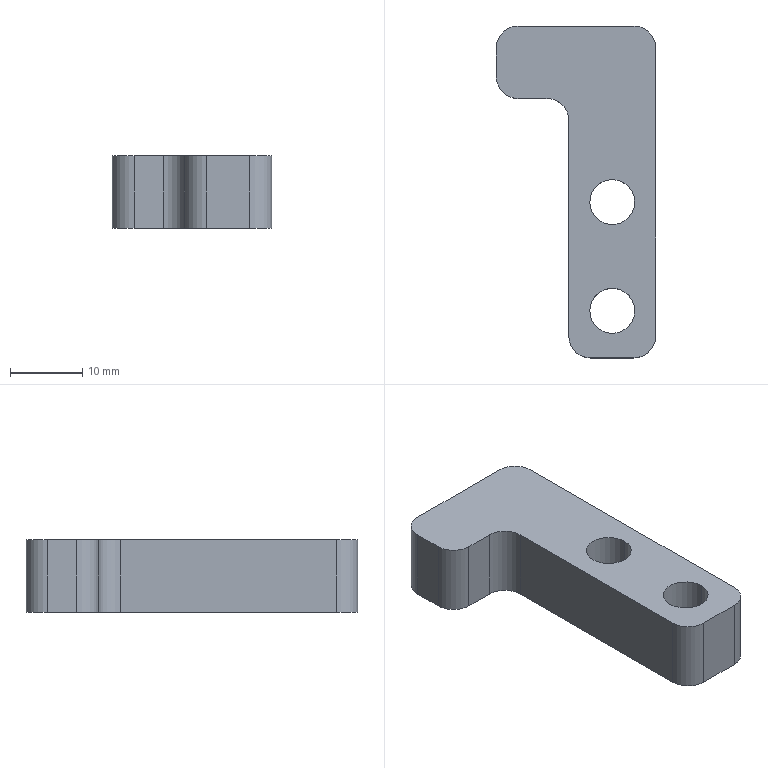CAM job | Mastercam | mm | 8 operations | part box 22 x 45.8 x 10
1. Facing | 23 - 63 平铣刀
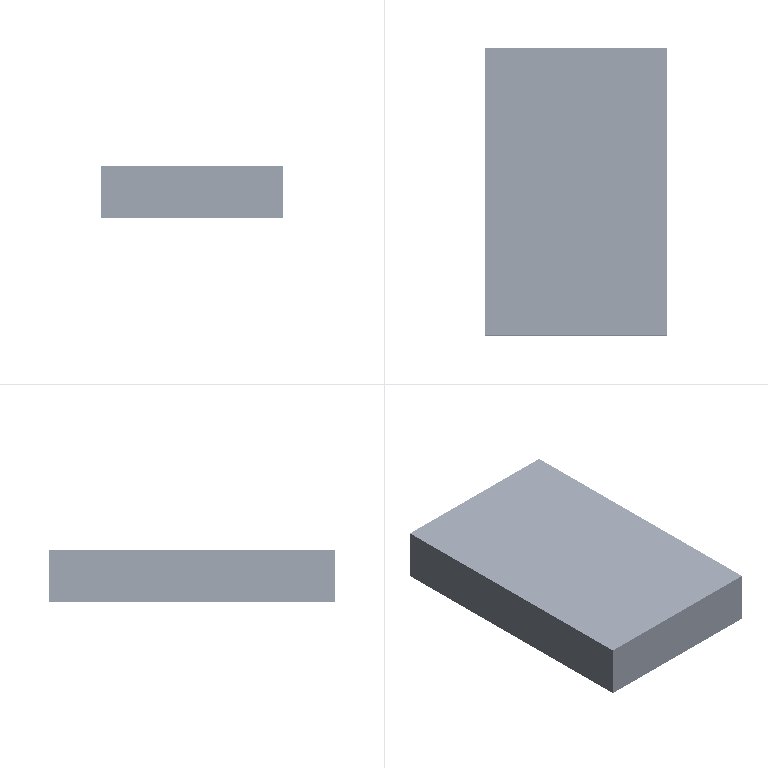2. 2D High Speed (2D Dynamic Mill) | 9 - 10 平铣刀
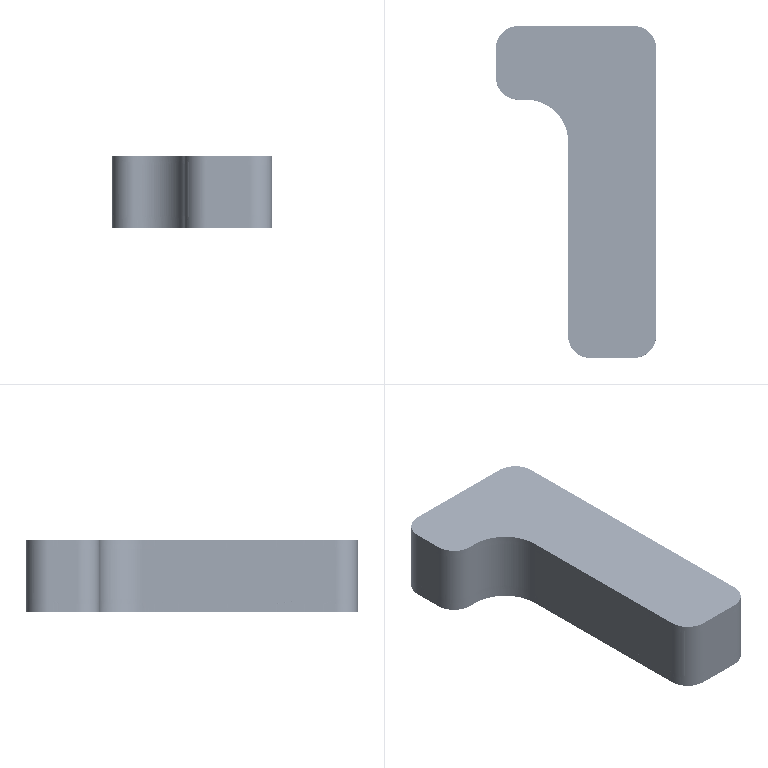3. Contour (Remachining) | 4 - 4 平铣刀
4. Contour (2D) | 4 - 4 平铣刀
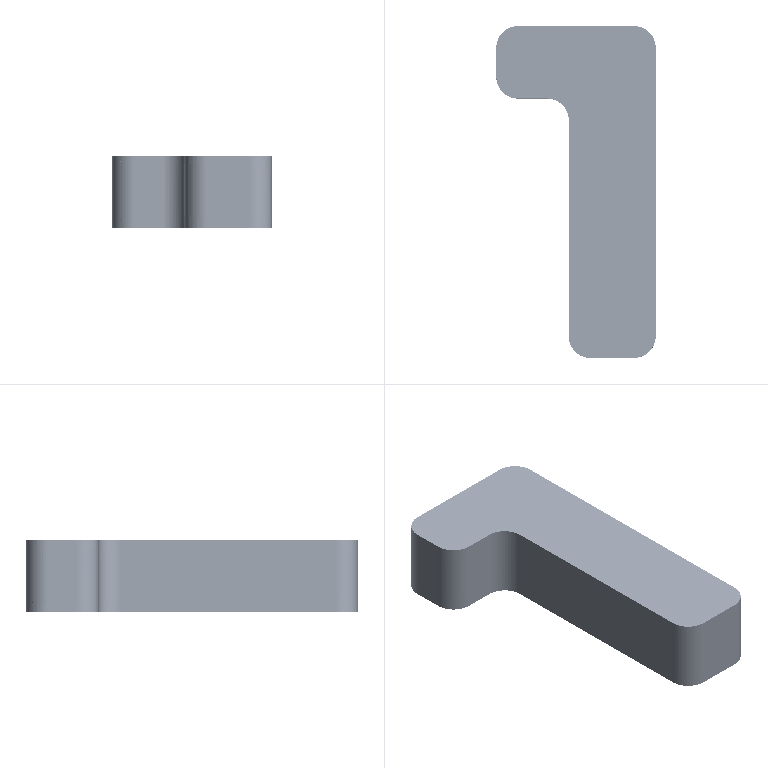5. Drill/Counterbore | 5 - 4 倒角刀
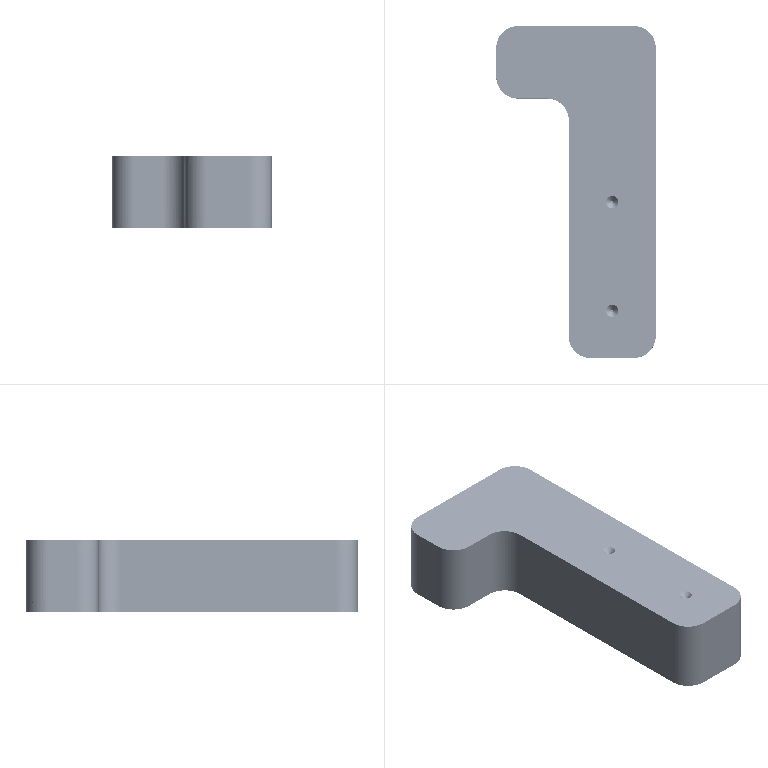6. Contour (2D chamfer) | 5 - 4 倒角刀
7. Facing | 9 - 10 平铣刀
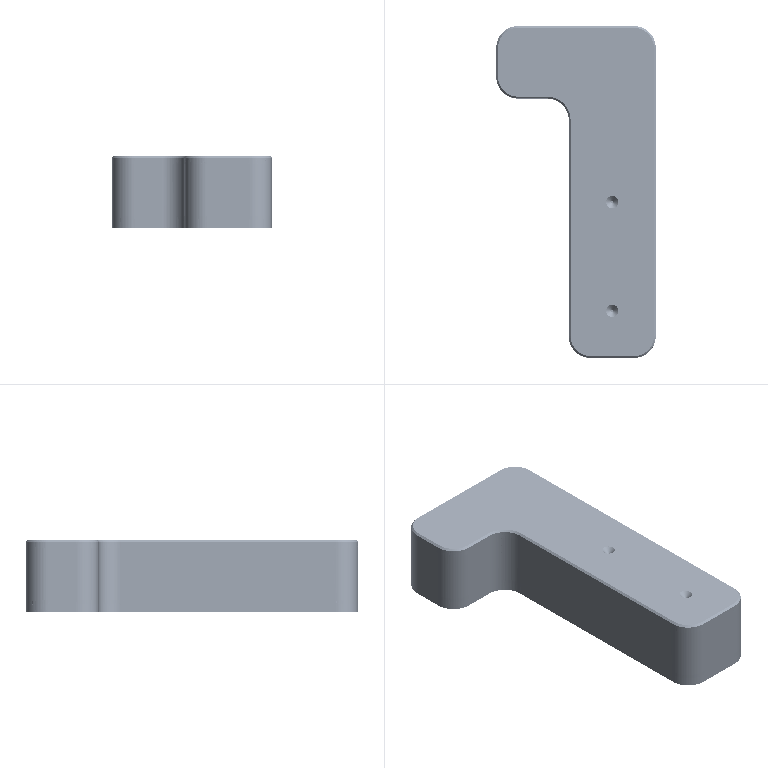8. Facing | 10 - 10 平铣刀